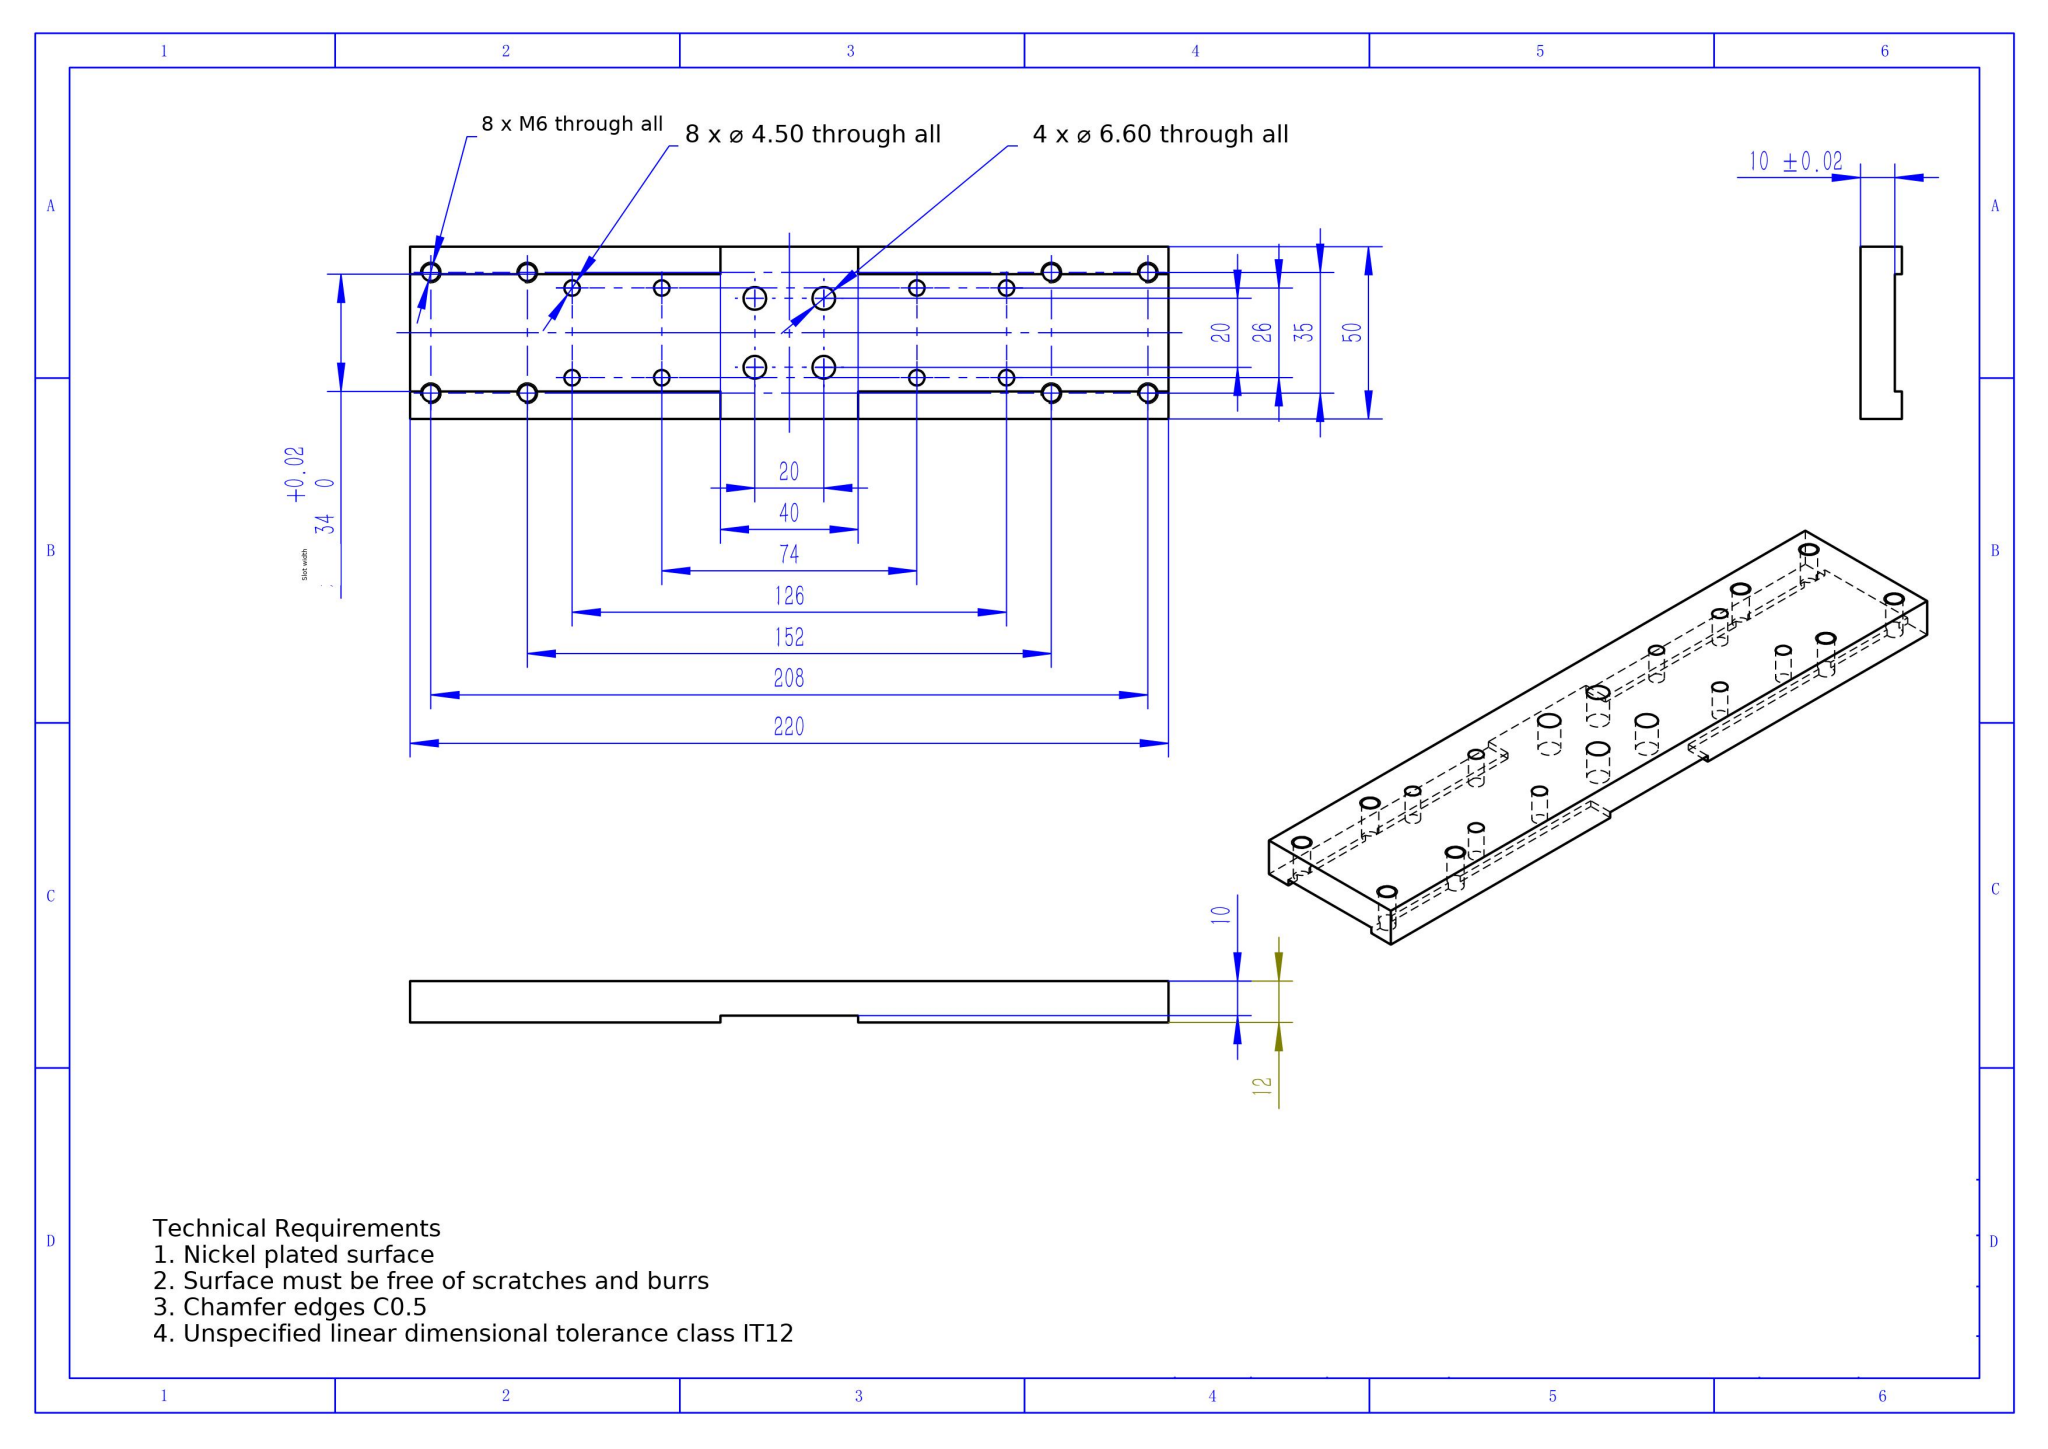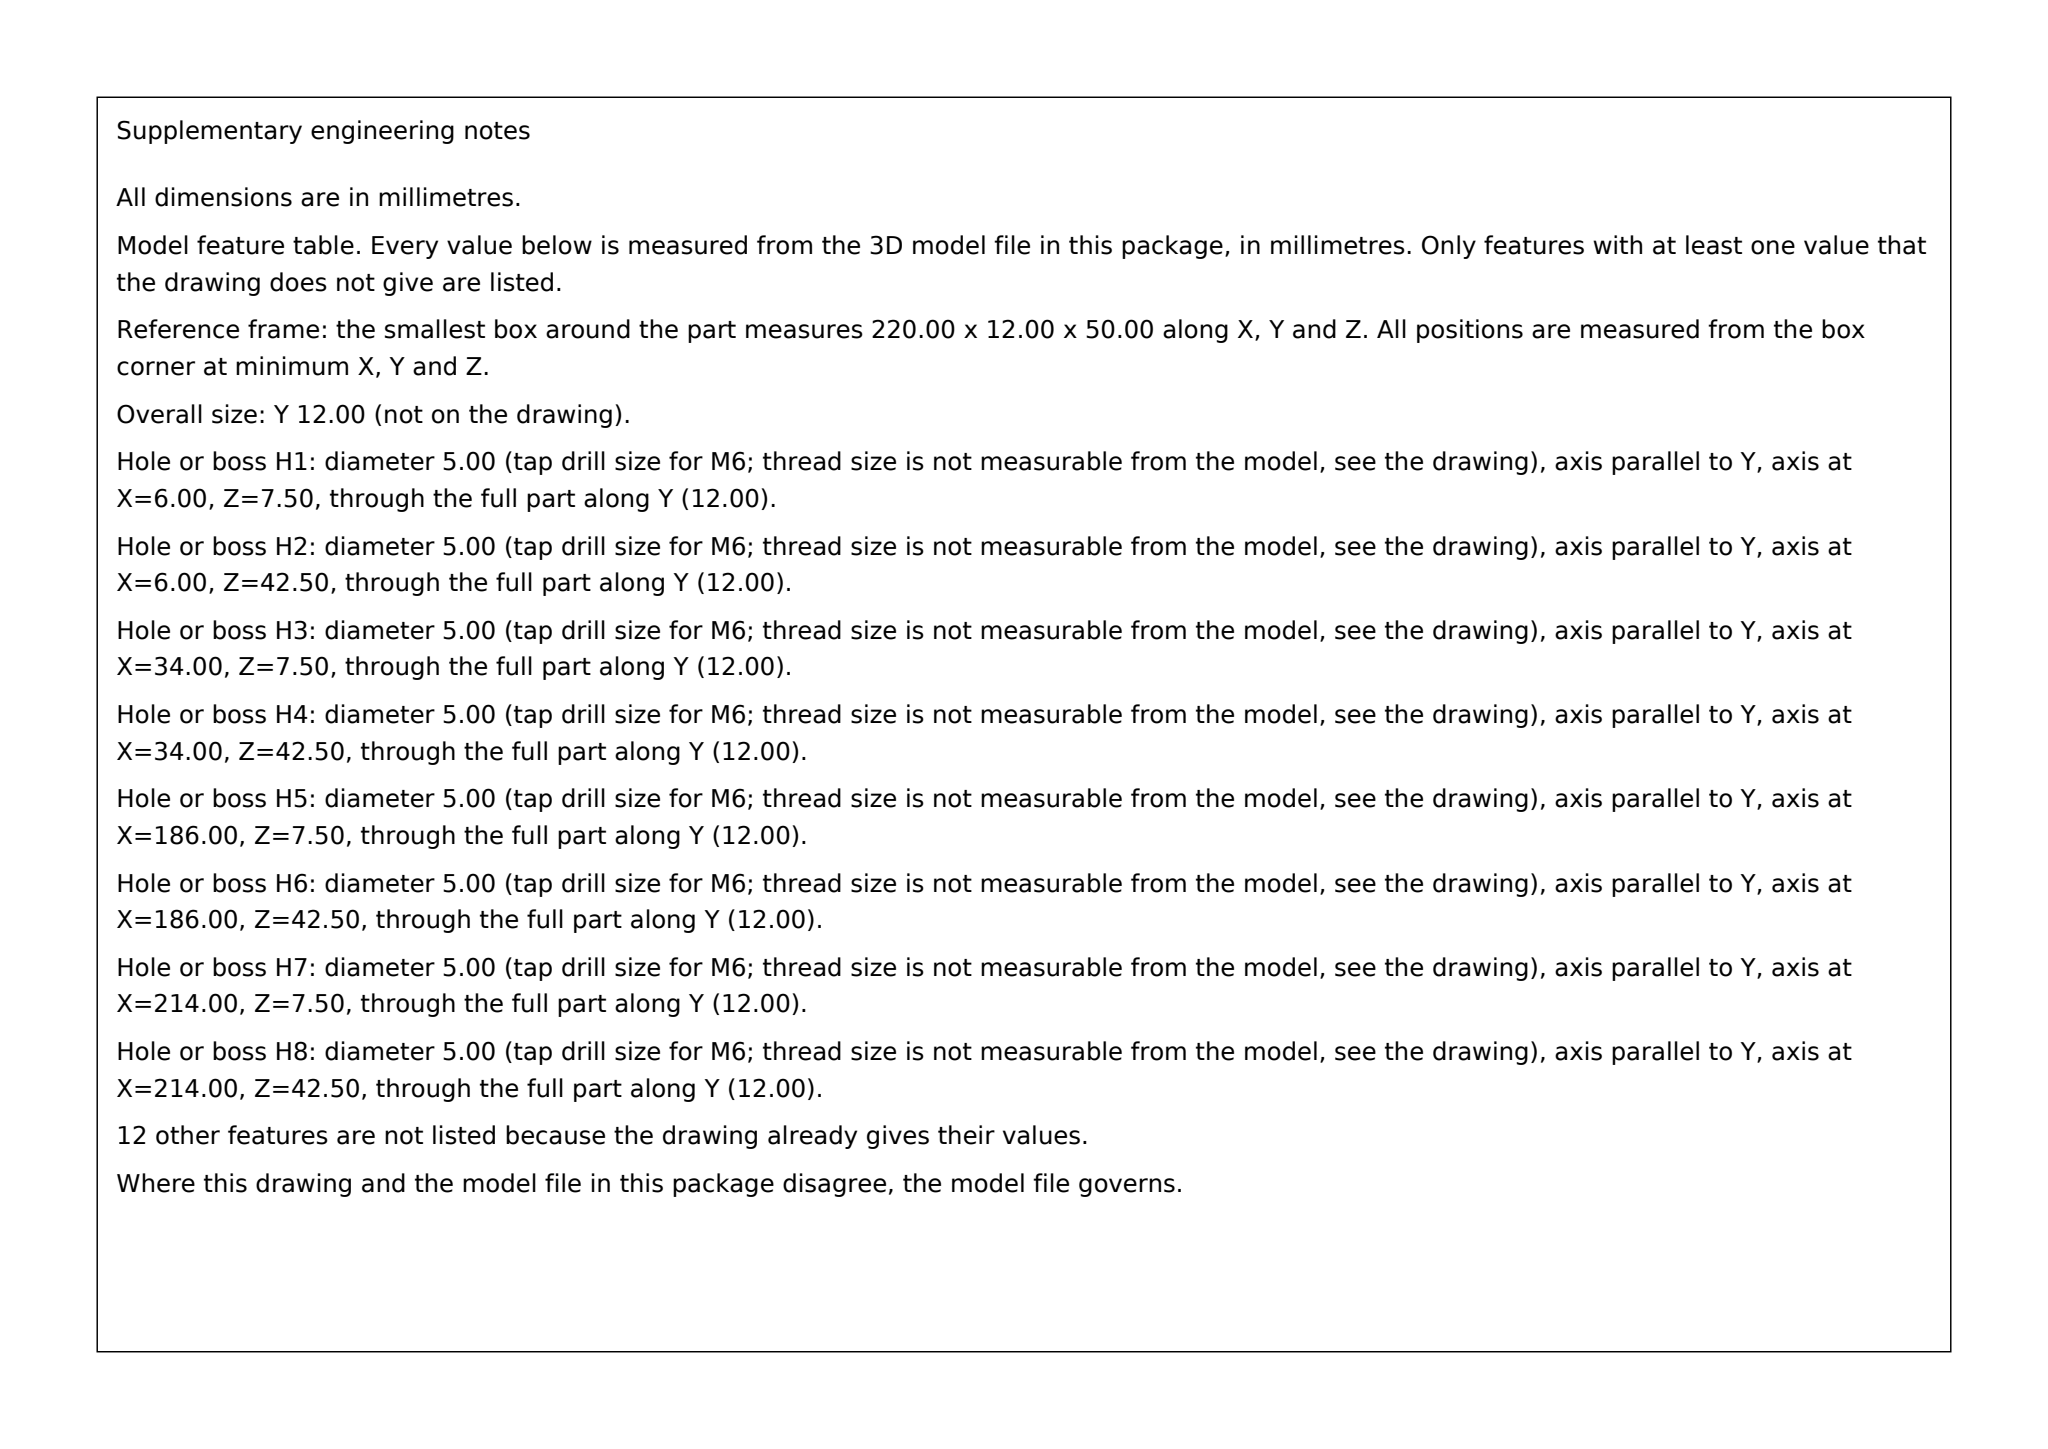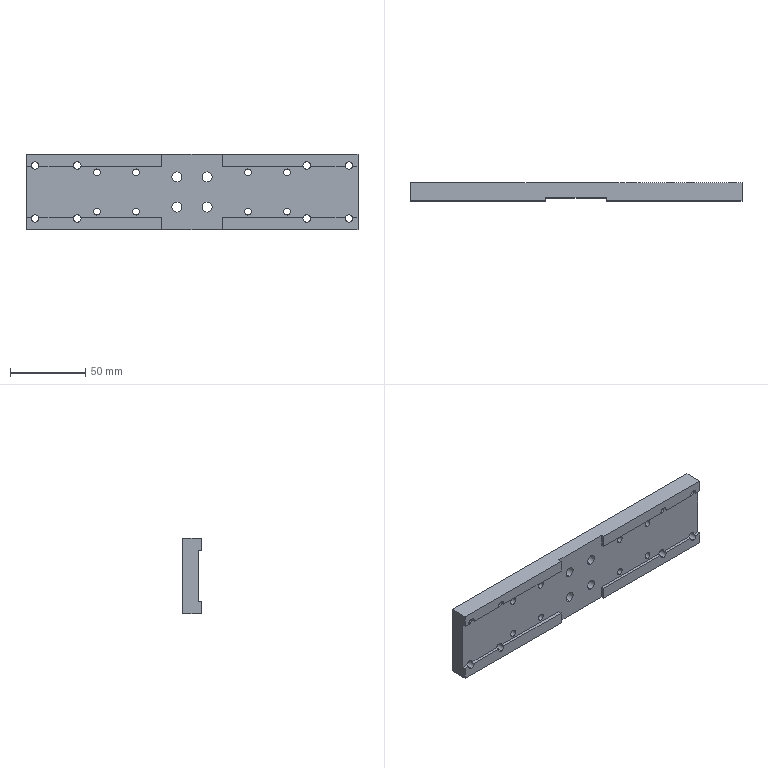Part | SolidWorks | mm | 1 solid | 66 faces | box 220 x 12 x 50 mm | volume 111352 mm3 | cylinder 40 | plane 26 | commonest cylinder face diameters 5 x16 4.5 x16 6.6 x8
build123d program:
from build123d import *

# Parameters (mm, degrees)
SKETCH1_W            = 220
SKETCH1_H            = 50
BOSS_EXTRUDE1_DEPTH  = 12
M4_CLEARANCE_HOLE1_D = 4.5
SKETCH4_W            = 220
SKETCH4_H            = 34
CUT_EXTRUDE1_DEPTH   = 2
M6_TAPPED_HOLE2_D    = 5
SKETCH5_W            = 40
SKETCH5_H            = 50
CUT_EXTRUDE2_DEPTH   = 2
M6_CLEARANCE_HOLE1_D = 6.6


with BuildPart() as part:
    # Sketch1 → Boss-Extrude1 (new body)
    with BuildSketch(Plane(origin=(0, 0, 0), x_dir=(1, 0, 0), z_dir=(0, 1, 0))):
        Rectangle(SKETCH1_W, SKETCH1_H)
    extrude(amount=BOSS_EXTRUDE1_DEPTH)

    # M4 Clearance Hole1 (through all)
    with Locations(Plane(origin=(0, 12, 0), x_dir=(1, 0, 0), z_dir=(0, 1, 0))):
        with Locations((-63, 13), (-37, -13), (-63, -13), (-37, 13)):
            m4_clearance_hole1 = Hole(M4_CLEARANCE_HOLE1_D / 2)

    # Sketch4 → Cut-Extrude1 (cut)
    with BuildSketch(Plane.XZ):
        Rectangle(SKETCH4_W, SKETCH4_H)
    extrude(amount=-CUT_EXTRUDE1_DEPTH, mode=Mode.SUBTRACT)

    # M6 Tapped Hole2 (through all)
    with Locations(Plane(origin=(0, 12, 0), x_dir=(1, 0, 0), z_dir=(0, 1, 0))):
        with Locations((-104, 17.5), (-76, -17.5), (-104, -17.5), (-76, 17.5)):
            m6_tapped_hole2 = Hole(M6_TAPPED_HOLE2_D / 2)

    # Sketch5 → Cut-Extrude2 (cut)
    with BuildSketch(Plane.XZ):
        Rectangle(SKETCH5_W, SKETCH5_H)
    extrude(amount=-CUT_EXTRUDE2_DEPTH, mode=Mode.SUBTRACT)

    # M6 Clearance Hole1 (through all)
    with Locations(Plane(origin=(0, 2, 0), x_dir=(-1, 0, 0), z_dir=(0, -1, 0))):
        with Locations((-10, 10), (10, -10), (-10, -10), (10, 10)):
            Hole(M6_CLEARANCE_HOLE1_D / 2)

    # Mirror1: M4 Clearance Hole1, M6 Tapped Hole2 across plane
    add(m4_clearance_hole1.mirror(Plane(origin=(0, 0, 0), x_dir=(0, 0, 1), z_dir=(1, 0, 0))), mode=Mode.SUBTRACT)
    add(m6_tapped_hole2.mirror(Plane(origin=(0, 0, 0), x_dir=(0, 0, 1), z_dir=(1, 0, 0))), mode=Mode.SUBTRACT)


solid = part.part